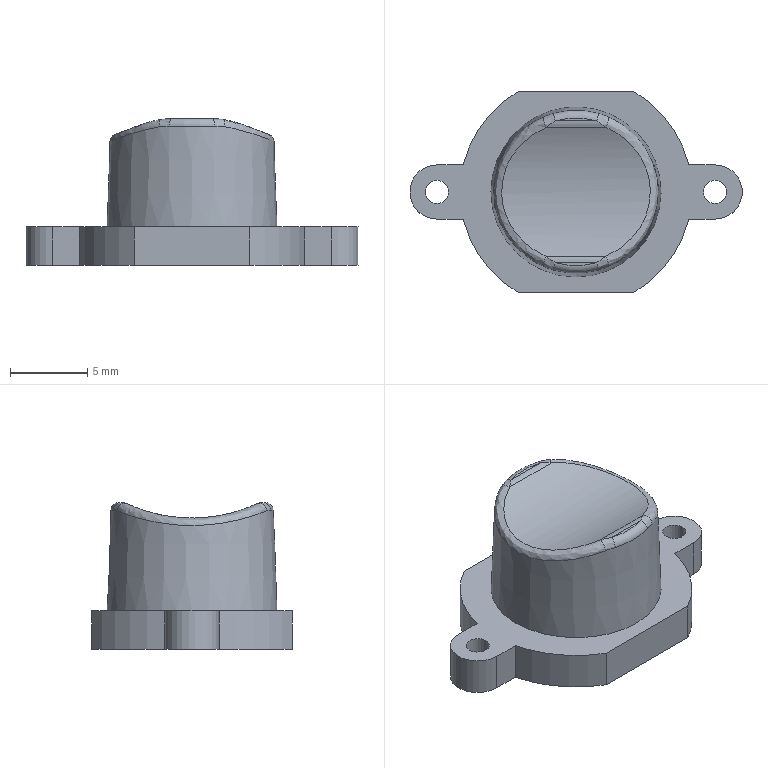Component | NX | ANNIU | 1 solid | 34 faces | volume 1030 mm3 | cylinder 13 | plane 12 | spline 6 | torus 2 | cone 1 | commonest cylinder face diameters 15 x4 2 x2 3.5 x2 1.5 x2 2.5 x2 20 x1